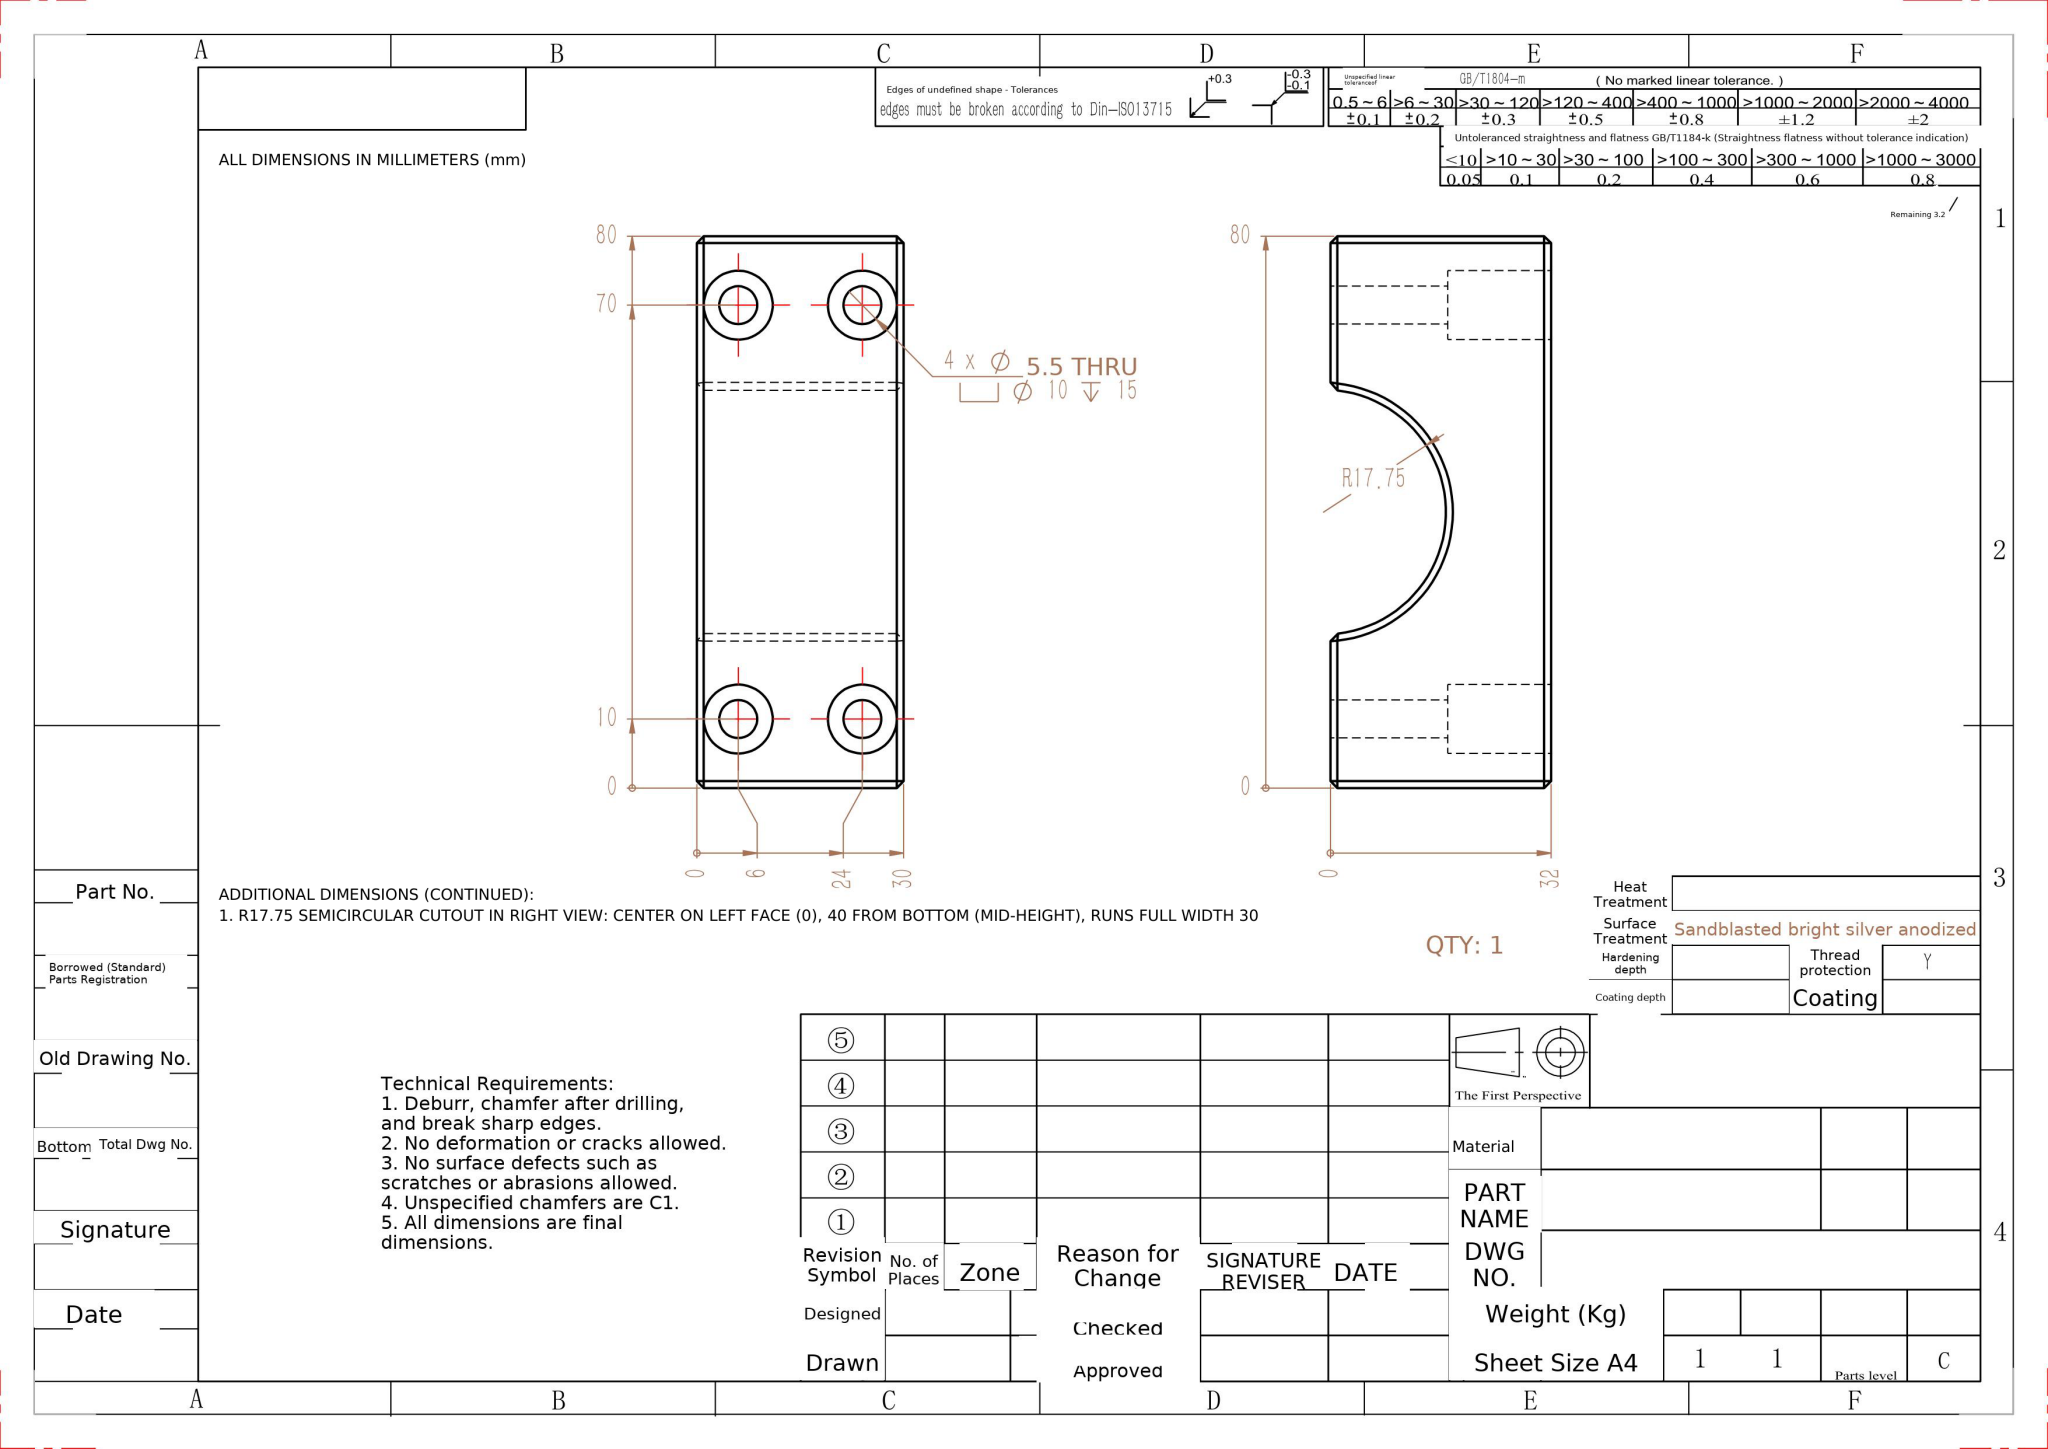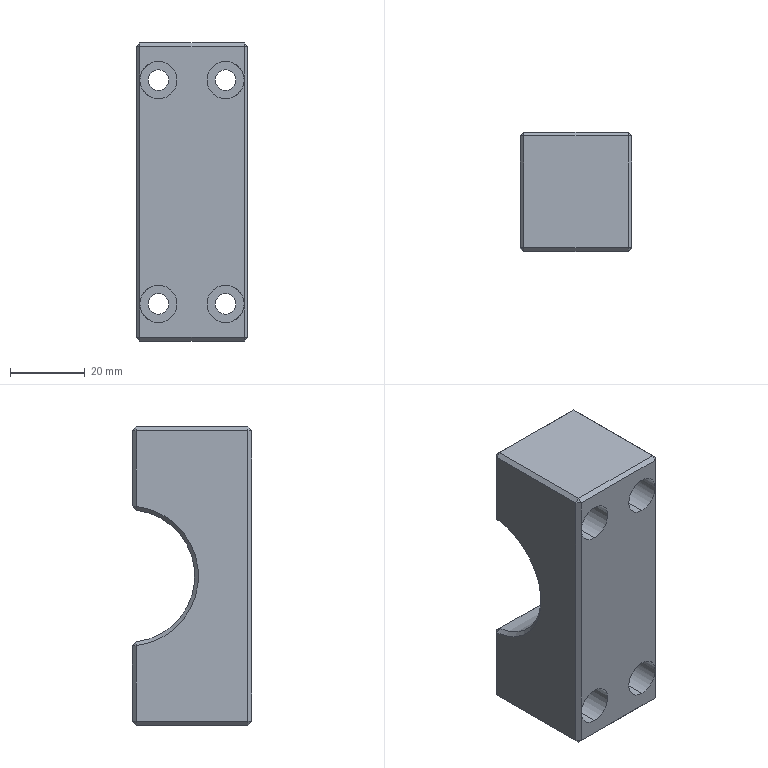Part | NX | mm | 1 solid | 58 faces | box 30 x 32 x 80 mm | volume 56362 mm3 | plane 39 | cylinder 17 | cone 2 | commonest cylinder face diameters 10 x8 5.5 x8 35.5 x1